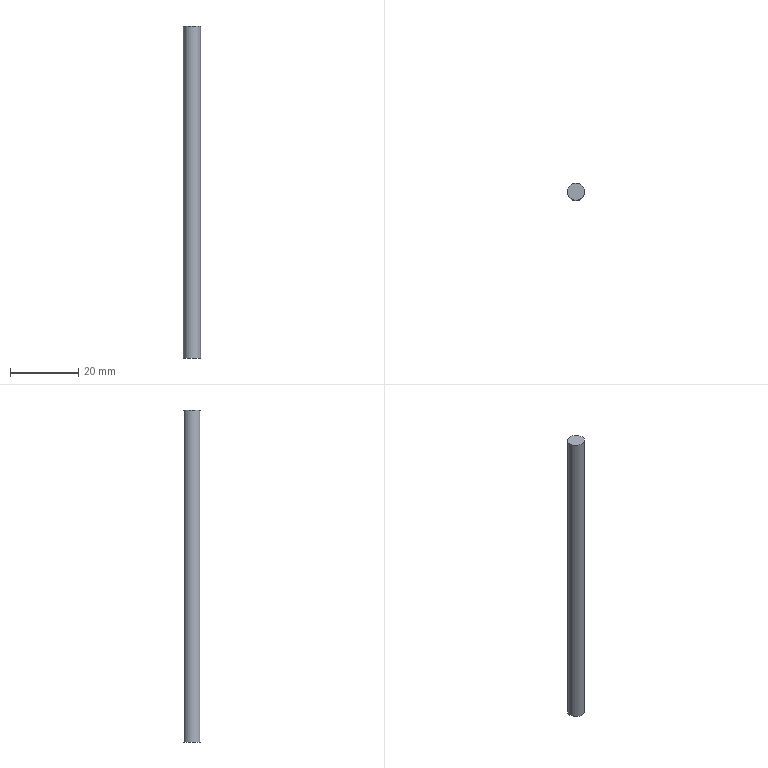Component | NX | SLIDE_POST | 1 solid | 3 faces | box 5 x 5 x 97 mm | volume 1905 mm3 | plane 2 | cylinder 1 | commonest cylinder face diameters 5 x1
STEP:
#1=CARTESIAN_POINT('',(0.,0.,0.));
#2=DIRECTION('',(0.,0.,1.));
#3=DIRECTION('',(1.,0.,0.));
#4=AXIS2_PLACEMENT_3D('',#1,#2,#3);
#5=CARTESIAN_POINT('',(-13.038,-24.899,31.833));
#6=VERTEX_POINT('',#5);
#7=CARTESIAN_POINT('',(-15.538,-24.899,31.833));
#8=DIRECTION('',(0.,0.,-1.));
#9=DIRECTION('',(1.,0.,0.));
#10=AXIS2_PLACEMENT_3D('',#7,#8,#9);
#11=CIRCLE('',#10,2.5);
#12=CARTESIAN_POINT('',(-15.538,-24.899,31.833));
#13=DIRECTION('',(0.,0.,1.));
#14=DIRECTION('',(1.,0.,0.));
#15=AXIS2_PLACEMENT_3D('',#12,#13,#14);
#16=PLANE('',#15);
#17=CARTESIAN_POINT('',(2.5,0.));
#18=CARTESIAN_POINT('',(2.5,-4.33));
#19=CARTESIAN_POINT('',(-1.25,-2.165));
#20=CARTESIAN_POINT('',(-5.,-0.));
#21=CARTESIAN_POINT('',(-1.25,2.165));
#22=CARTESIAN_POINT('',(2.5,4.33));
#23=CARTESIAN_POINT('',(2.5,0.));
#24=(BOUNDED_CURVE()B_SPLINE_CURVE(2,(#17,#18,#19,#20,#21,#22,#23),.UNSPECIFIED.,.T.,.F.)B_SPLINE_CURVE_WITH_KNOTS((1,2,2,2,2,1),(-2.094,0.,2.094,4.189,6.283,8.378),.UNSPECIFIED.)CURVE()GEOMETRIC_REPRESENTATION_ITEM()RATIONAL_B_SPLINE_CURVE((1.,0.5,1.,0.5,1.,0.5,1.))REPRESENTATION_ITEM(''));
#25=(GEOMETRIC_REPRESENTATION_CONTEXT(2)PARAMETRIC_REPRESENTATION_CONTEXT()REPRESENTATION_CONTEXT('',''));
#26=DEFINITIONAL_REPRESENTATION('',(#24),#25);
#27=PCURVE('',#16,#26);
#28=CARTESIAN_POINT('',(-15.538,-24.899,-65.167));
#29=DIRECTION('',(0.,0.,1.));
#30=DIRECTION('',(1.,0.,0.));
#31=AXIS2_PLACEMENT_3D('',#28,#29,#30);
#32=CYLINDRICAL_SURFACE('',#31,2.5);
#33=CARTESIAN_POINT('',(6.283,97.));
#34=DIRECTION('',(-1.,0.));
#35=VECTOR('',#34,1.);
#36=LINE('',#33,#35);
#37=(GEOMETRIC_REPRESENTATION_CONTEXT(2)PARAMETRIC_REPRESENTATION_CONTEXT()REPRESENTATION_CONTEXT('',''));
#38=DEFINITIONAL_REPRESENTATION('',(#36),#37);
#39=PCURVE('',#32,#38);
#40=SURFACE_CURVE('',#11,(#27,#39),.PCURVE_S1.);
#41=EDGE_CURVE('',#6,#6,#40,.T.);
#42=ORIENTED_EDGE('',*,*,#41,.F.);
#43=EDGE_LOOP('',(#42));
#44=FACE_BOUND('',#43,.T.);
#45=ADVANCED_FACE('',(#44),#16,.T.);
#46=CARTESIAN_POINT('',(-13.038,-24.899,-65.167));
#47=VERTEX_POINT('',#46);
#48=CARTESIAN_POINT('',(-15.538,-24.899,-65.167));
#49=DIRECTION('',(0.,0.,1.));
#50=DIRECTION('',(1.,0.,0.));
#51=AXIS2_PLACEMENT_3D('',#48,#49,#50);
#52=CIRCLE('',#51,2.5);
#53=CARTESIAN_POINT('',(-15.538,-24.899,-65.167));
#54=DIRECTION('',(0.,0.,-1.));
#55=DIRECTION('',(-1.,0.,0.));
#56=AXIS2_PLACEMENT_3D('',#53,#54,#55);
#57=PLANE('',#56);
#58=CARTESIAN_POINT('',(-2.5,0.));
#59=CARTESIAN_POINT('',(-2.5,4.33));
#60=CARTESIAN_POINT('',(1.25,2.165));
#61=CARTESIAN_POINT('',(5.,0.));
#62=CARTESIAN_POINT('',(1.25,-2.165));
#63=CARTESIAN_POINT('',(-2.5,-4.33));
#64=CARTESIAN_POINT('',(-2.5,0.));
#65=(BOUNDED_CURVE()B_SPLINE_CURVE(2,(#58,#59,#60,#61,#62,#63,#64),.UNSPECIFIED.,.T.,.F.)B_SPLINE_CURVE_WITH_KNOTS((1,2,2,2,2,1),(-2.094,0.,2.094,4.189,6.283,8.378),.UNSPECIFIED.)CURVE()GEOMETRIC_REPRESENTATION_ITEM()RATIONAL_B_SPLINE_CURVE((1.,0.5,1.,0.5,1.,0.5,1.))REPRESENTATION_ITEM(''));
#66=(GEOMETRIC_REPRESENTATION_CONTEXT(2)PARAMETRIC_REPRESENTATION_CONTEXT()REPRESENTATION_CONTEXT('',''));
#67=DEFINITIONAL_REPRESENTATION('',(#65),#66);
#68=PCURVE('',#57,#67);
#69=CARTESIAN_POINT('',(0.,0.));
#70=DIRECTION('',(1.,0.));
#71=VECTOR('',#70,1.);
#72=LINE('',#69,#71);
#73=(GEOMETRIC_REPRESENTATION_CONTEXT(2)PARAMETRIC_REPRESENTATION_CONTEXT()REPRESENTATION_CONTEXT('',''));
#74=DEFINITIONAL_REPRESENTATION('',(#72),#73);
#75=PCURVE('',#32,#74);
#76=SURFACE_CURVE('',#52,(#68,#75),.PCURVE_S1.);
#77=EDGE_CURVE('',#47,#47,#76,.T.);
#78=ORIENTED_EDGE('',*,*,#77,.F.);
#79=EDGE_LOOP('',(#78));
#80=FACE_BOUND('',#79,.T.);
#81=ADVANCED_FACE('',(#80),#57,.T.);
#82=ORIENTED_EDGE('',*,*,#41,.T.);
#83=CARTESIAN_POINT('',(-13.038,-24.899,-65.167));
#84=CARTESIAN_POINT('',(-13.038,-24.899,31.833));
#85=B_SPLINE_CURVE_WITH_KNOTS('',1,(#83,#84),.UNSPECIFIED.,.F.,.F.,(2,2),(0.,97.),.PIECEWISE_BEZIER_KNOTS.);
#86=CARTESIAN_POINT('',(0.,0.));
#87=DIRECTION('',(0.,1.));
#88=VECTOR('',#87,1.);
#89=LINE('',#86,#88);
#90=(GEOMETRIC_REPRESENTATION_CONTEXT(2)PARAMETRIC_REPRESENTATION_CONTEXT()REPRESENTATION_CONTEXT('',''));
#91=DEFINITIONAL_REPRESENTATION('',(#89),#90);
#92=PCURVE('',#32,#91);
#93=CARTESIAN_POINT('',(6.283,0.));
#94=DIRECTION('',(0.,1.));
#95=VECTOR('',#94,1.);
#96=LINE('',#93,#95);
#97=(GEOMETRIC_REPRESENTATION_CONTEXT(2)PARAMETRIC_REPRESENTATION_CONTEXT()REPRESENTATION_CONTEXT('',''));
#98=DEFINITIONAL_REPRESENTATION('',(#96),#97);
#99=PCURVE('',#32,#98);
#100=SEAM_CURVE('',#85,(#92,#99),.PCURVE_S1.);
#101=EDGE_CURVE('',#47,#6,#100,.T.);
#102=ORIENTED_EDGE('',*,*,#101,.F.);
#103=ORIENTED_EDGE('',*,*,#77,.T.);
#104=ORIENTED_EDGE('',*,*,#101,.T.);
#105=EDGE_LOOP('',(#82,#102,#103,#104));
#106=FACE_BOUND('',#105,.T.);
#107=ADVANCED_FACE('',(#106),#32,.T.);
#108=CLOSED_SHELL('',(#45,#81,#107));
#109=MANIFOLD_SOLID_BREP('',#108);
#110=(LENGTH_UNIT()NAMED_UNIT(*)SI_UNIT(.MILLI.,.METRE.));
#111=UNCERTAINTY_MEASURE_WITH_UNIT(LENGTH_MEASURE(0.00001),#110,'','');
#112=(NAMED_UNIT(*)PLANE_ANGLE_UNIT()SI_UNIT($,.RADIAN.));
#113=(NAMED_UNIT(*)SI_UNIT($,.STERADIAN.)SOLID_ANGLE_UNIT());
#114=(GEOMETRIC_REPRESENTATION_CONTEXT(3)GLOBAL_UNCERTAINTY_ASSIGNED_CONTEXT((#111))GLOBAL_UNIT_ASSIGNED_CONTEXT((#110,#112,#113))REPRESENTATION_CONTEXT('',''));
#115=ADVANCED_BREP_SHAPE_REPRESENTATION('',(#4,#109),#114);